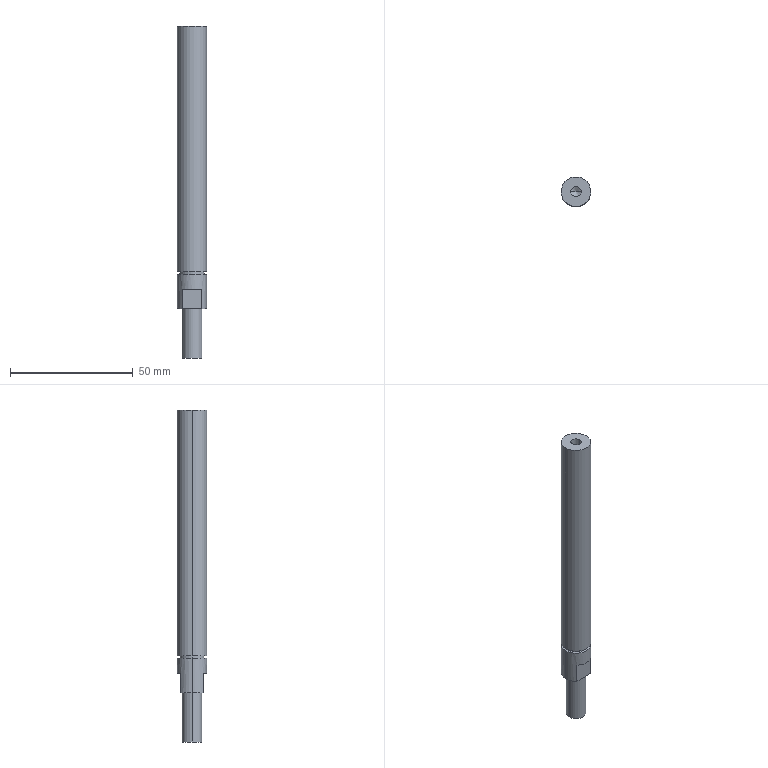Component | SolidWorks | GuideWheelAssembly2-1_RollerAxis1-1 | 1 solid | 21 faces | box 12 x 12 x 135 mm | volume 13669 mm3 | cylinder 10 | plane 9 | cone 2 | commonest cylinder face diameters 12 x4 8 x2 10 x2 4.2 x2
build123d program:
from build123d import *

# Parameters (mm, degrees)
SKETCH1_R             = 6
BOSS_EXTRUDE1_DEPTH   = 115
SKETCH3_R             = 4
BOSS_EXTRUDE2_DEPTH   = 20
CUT_EXTRUDE7_START    = -8
CUT_EXTRUDE7_DEPTH    = 8
M5_TAPPED_HOLE1_D     = 4.2
M5_TAPPED_HOLE1_DEPTH = 12.4
M5_TAPPED_HOLE1_TIP   = 1.262
SKETCH20_W            = 1
SKETCH20_H            = 1


with BuildPart() as part:
    # Sketch1 → Boss-Extrude1 (new body)
    with BuildSketch(Plane(origin=(0, 0, 0), x_dir=(1, 0, 0), z_dir=(0, 1, 0))):
        with Locations(Location((0, 0, 0), (0, 0, 270))):
            Circle(SKETCH1_R)
    extrude(amount=BOSS_EXTRUDE1_DEPTH)

    # Sketch3 → Boss-Extrude2 (add)
    with BuildSketch(Plane(origin=(0, 115, 0), x_dir=(1, 0, 0), z_dir=(0, 1, 0))):
        with Locations(Location((0, 0, 0), (0, 0, 270))):
            Circle(SKETCH3_R)
    extrude(amount=BOSS_EXTRUDE2_DEPTH)

    # Sketch17 → Cut-Extrude7 (cut)
    with BuildSketch(Plane(origin=(0, 115, 0), x_dir=(1, 0, 0), z_dir=(0, 1, 0)).offset(CUT_EXTRUDE7_START)):
        with BuildLine():
            Line((-4.5, 3.969), (-4.5, -3.969))
            ThreePointArc((-4.5, -3.969), (-6, 0), (-4.5, 3.969))
        make_face()
        with BuildLine():
            Line((4.5, 3.969), (4.5, -3.969))
            ThreePointArc((4.5, -3.969), (6, 0), (4.5, 3.969))
        make_face()
    extrude(amount=CUT_EXTRUDE7_DEPTH, mode=Mode.SUBTRACT)

    # M5 Tapped Hole1
    with Locations(Plane(origin=(0, 0, 0), x_dir=(-1, 0, 0), z_dir=(0, -1, 0))):
        with Locations((0, 0)):
            Hole(M5_TAPPED_HOLE1_D / 2, depth=M5_TAPPED_HOLE1_DEPTH)
            with Locations((0, 0, -(M5_TAPPED_HOLE1_DEPTH + M5_TAPPED_HOLE1_TIP / 2))):  # 118° drill point
                Cone(0, M5_TAPPED_HOLE1_D / 2, M5_TAPPED_HOLE1_TIP, mode=Mode.SUBTRACT)

    # Sketch20 → Cut-Revolve1 (revolve, cut)
    with BuildSketch(Plane(origin=(0, 0, 0), x_dir=(0, 0, -1), z_dir=(1, 0, 0)), mode=Mode.PRIVATE) as cut_revolve1_sk:
        with Locations((5.5, 100.5)):
            Rectangle(SKETCH20_W, SKETCH20_H)
    revolve(cut_revolve1_sk.sketch.rotate(Axis((0, 135, 0), (0, -1, 0)), 311.41), axis=Axis((0, 135, 0), (0, -1, 0)), mode=Mode.SUBTRACT)


solid = part.part

# Placed as in the assembly
solid = solid.moved(Location((-479.97, -65, 117), (-90, 90, 0)))
STEP:
#1=CARTESIAN_POINT('',(-18.66,-2.559,0.07874));
#2=VERTEX_POINT('',#1);
#3=CARTESIAN_POINT('',(-18.74,-2.736,0.07874));
#4=VERTEX_POINT('',#3);
#5=CARTESIAN_POINT('',(-18.896,-2.559,0.07874));
#6=DIRECTION('',(0.,0.,-1.));
#7=DIRECTION('',(1.,0.,-0.));
#8=AXIS2_PLACEMENT_3D('',#5,#6,#7);
#9=CIRCLE('',#8,0.2362);
#10=EDGE_CURVE('',#2,#4,#9,.T.);
#11=ORIENTED_EDGE('',*,*,#10,.F.);
#12=CARTESIAN_POINT('',(-18.66,-2.559,0.6299));
#13=VERTEX_POINT('',#12);
#14=CARTESIAN_POINT('',(-18.66,-2.559,0.07874));
#15=DIRECTION('',(-0.,-0.,1.));
#16=VECTOR('',#15,39.37);
#17=LINE('',#14,#16);
#18=EDGE_CURVE('',#2,#13,#17,.T.);
#19=ORIENTED_EDGE('',*,*,#18,.T.);
#20=CARTESIAN_POINT('',(-19.133,-2.559,0.6299));
#21=VERTEX_POINT('',#20);
#22=CARTESIAN_POINT('',(-18.896,-2.559,0.6299));
#23=DIRECTION('',(0.,0.,-1.));
#24=DIRECTION('',(1.,0.,0.));
#25=AXIS2_PLACEMENT_3D('',#22,#23,#24);
#26=CIRCLE('',#25,0.2362);
#27=EDGE_CURVE('',#13,#21,#26,.T.);
#28=ORIENTED_EDGE('',*,*,#27,.T.);
#29=CARTESIAN_POINT('',(-19.133,-2.559,0.07874));
#30=VERTEX_POINT('',#29);
#31=CARTESIAN_POINT('',(-19.133,-2.559,0.07874));
#32=DIRECTION('',(-0.,-0.,1.));
#33=VECTOR('',#32,39.37);
#34=LINE('',#31,#33);
#35=EDGE_CURVE('',#30,#21,#34,.T.);
#36=ORIENTED_EDGE('',*,*,#35,.F.);
#37=CARTESIAN_POINT('',(-19.053,-2.736,0.07874));
#38=VERTEX_POINT('',#37);
#39=CARTESIAN_POINT('',(-18.896,-2.559,0.07874));
#40=DIRECTION('',(0.,0.,-1.));
#41=DIRECTION('',(1.,0.,-0.));
#42=AXIS2_PLACEMENT_3D('',#39,#40,#41);
#43=CIRCLE('',#42,0.2362);
#44=EDGE_CURVE('',#38,#30,#43,.T.);
#45=ORIENTED_EDGE('',*,*,#44,.F.);
#46=CARTESIAN_POINT('',(-19.053,-2.736,0.3937));
#47=VERTEX_POINT('',#46);
#48=CARTESIAN_POINT('',(-19.053,-2.736,0.3937));
#49=DIRECTION('',(0.,0.,-1.));
#50=VECTOR('',#49,39.37);
#51=LINE('',#48,#50);
#52=EDGE_CURVE('',#47,#38,#51,.T.);
#53=ORIENTED_EDGE('',*,*,#52,.F.);
#54=CARTESIAN_POINT('',(-18.74,-2.736,0.3937));
#55=VERTEX_POINT('',#54);
#56=CARTESIAN_POINT('',(-18.896,-2.559,0.3937));
#57=DIRECTION('',(0.,0.,-1.));
#58=DIRECTION('',(1.,0.,0.));
#59=AXIS2_PLACEMENT_3D('',#56,#57,#58);
#60=CIRCLE('',#59,0.2362);
#61=EDGE_CURVE('',#55,#47,#60,.T.);
#62=ORIENTED_EDGE('',*,*,#61,.F.);
#63=CARTESIAN_POINT('',(-18.74,-2.736,0.3937));
#64=DIRECTION('',(0.,0.,-1.));
#65=VECTOR('',#64,39.37);
#66=LINE('',#63,#65);
#67=EDGE_CURVE('',#55,#4,#66,.T.);
#68=ORIENTED_EDGE('',*,*,#67,.T.);
#69=EDGE_LOOP('',(#11,#19,#28,#36,#45,#53,#62,#68));
#70=FACE_OUTER_BOUND('',#69,.T.);
#71=CARTESIAN_POINT('',(-18.896,-2.559,0.07874));
#72=DIRECTION('',(-0.,-0.,1.));
#73=DIRECTION('',(-1.,0.,0.));
#74=AXIS2_PLACEMENT_3D('',#71,#72,#73);
#75=CYLINDRICAL_SURFACE('',#74,0.2362);
#76=ADVANCED_FACE('',(#70),#75,.T.);
#77=CARTESIAN_POINT('',(-18.739,-2.559,-0.7087));
#78=VERTEX_POINT('',#77);
#79=CARTESIAN_POINT('',(-19.054,-2.559,-0.7087));
#80=VERTEX_POINT('',#79);
#81=CARTESIAN_POINT('',(-18.896,-2.559,-0.7087));
#82=DIRECTION('',(0.,0.,-1.));
#83=DIRECTION('',(1.,0.,0.));
#84=AXIS2_PLACEMENT_3D('',#81,#82,#83);
#85=CIRCLE('',#84,0.1575);
#86=EDGE_CURVE('',#78,#80,#85,.T.);
#87=ORIENTED_EDGE('',*,*,#86,.F.);
#88=CARTESIAN_POINT('',(-18.739,-2.559,0.07874));
#89=VERTEX_POINT('',#88);
#90=CARTESIAN_POINT('',(-18.739,-2.559,-0.7087));
#91=DIRECTION('',(-0.,-0.,1.));
#92=VECTOR('',#91,39.37);
#93=LINE('',#90,#92);
#94=EDGE_CURVE('',#78,#89,#93,.T.);
#95=ORIENTED_EDGE('',*,*,#94,.T.);
#96=CARTESIAN_POINT('',(-19.054,-2.559,0.07874));
#97=VERTEX_POINT('',#96);
#98=CARTESIAN_POINT('',(-18.896,-2.559,0.07874));
#99=DIRECTION('',(0.,0.,-1.));
#100=DIRECTION('',(1.,0.,-0.));
#101=AXIS2_PLACEMENT_3D('',#98,#99,#100);
#102=CIRCLE('',#101,0.1575);
#103=EDGE_CURVE('',#89,#97,#102,.T.);
#104=ORIENTED_EDGE('',*,*,#103,.T.);
#105=CARTESIAN_POINT('',(-19.054,-2.559,-0.7087));
#106=DIRECTION('',(-0.,-0.,1.));
#107=VECTOR('',#106,39.37);
#108=LINE('',#105,#107);
#109=EDGE_CURVE('',#80,#97,#108,.T.);
#110=ORIENTED_EDGE('',*,*,#109,.F.);
#111=EDGE_LOOP('',(#87,#95,#104,#110));
#112=FACE_OUTER_BOUND('',#111,.T.);
#113=CARTESIAN_POINT('',(-18.896,-2.559,-0.7087));
#114=DIRECTION('',(-0.,-0.,1.));
#115=DIRECTION('',(-1.,0.,0.));
#116=AXIS2_PLACEMENT_3D('',#113,#114,#115);
#117=CYLINDRICAL_SURFACE('',#116,0.1575);
#118=ADVANCED_FACE('',(#112),#117,.T.);
#119=CARTESIAN_POINT('',(-18.7,-2.559,0.6693));
#120=VERTEX_POINT('',#119);
#121=CARTESIAN_POINT('',(-19.093,-2.559,0.6693));
#122=VERTEX_POINT('',#121);
#123=CARTESIAN_POINT('',(-18.896,-2.559,0.6693));
#124=DIRECTION('',(0.,0.,-1.));
#125=DIRECTION('',(1.,0.,0.));
#126=AXIS2_PLACEMENT_3D('',#123,#124,#125);
#127=CIRCLE('',#126,0.1969);
#128=EDGE_CURVE('',#120,#122,#127,.T.);
#129=ORIENTED_EDGE('',*,*,#128,.T.);
#130=CARTESIAN_POINT('',(-19.093,-2.559,0.6299));
#131=VERTEX_POINT('',#130);
#132=CARTESIAN_POINT('',(-19.093,-2.559,-0.7087));
#133=DIRECTION('',(0.,0.,-1.));
#134=VECTOR('',#133,39.37);
#135=LINE('',#132,#134);
#136=EDGE_CURVE('',#122,#131,#135,.T.);
#137=ORIENTED_EDGE('',*,*,#136,.T.);
#138=CARTESIAN_POINT('',(-18.7,-2.559,0.6299));
#139=VERTEX_POINT('',#138);
#140=CARTESIAN_POINT('',(-18.896,-2.559,0.6299));
#141=DIRECTION('',(0.,0.,-1.));
#142=DIRECTION('',(1.,0.,0.));
#143=AXIS2_PLACEMENT_3D('',#140,#141,#142);
#144=CIRCLE('',#143,0.1969);
#145=EDGE_CURVE('',#139,#131,#144,.T.);
#146=ORIENTED_EDGE('',*,*,#145,.F.);
#147=CARTESIAN_POINT('',(-18.7,-2.559,-0.7087));
#148=DIRECTION('',(0.,0.,-1.));
#149=VECTOR('',#148,39.37);
#150=LINE('',#147,#149);
#151=EDGE_CURVE('',#120,#139,#150,.T.);
#152=ORIENTED_EDGE('',*,*,#151,.F.);
#153=EDGE_LOOP('',(#129,#137,#146,#152));
#154=FACE_OUTER_BOUND('',#153,.T.);
#155=CARTESIAN_POINT('',(-18.896,-2.559,-0.7087));
#156=DIRECTION('',(0.,0.,-1.));
#157=DIRECTION('',(1.,0.,0.));
#158=AXIS2_PLACEMENT_3D('',#155,#156,#157);
#159=CYLINDRICAL_SURFACE('',#158,0.1969);
#160=ADVANCED_FACE('',(#154),#159,.T.);
#161=CARTESIAN_POINT('',(-18.814,-2.559,4.118));
#162=VERTEX_POINT('',#161);
#163=CARTESIAN_POINT('',(-18.979,-2.559,4.118));
#164=VERTEX_POINT('',#163);
#165=CARTESIAN_POINT('',(-18.896,-2.559,4.118));
#166=DIRECTION('',(-0.,-0.,1.));
#167=DIRECTION('',(-1.,0.,0.));
#168=AXIS2_PLACEMENT_3D('',#165,#166,#167);
#169=CIRCLE('',#168,0.08268);
#170=EDGE_CURVE('',#162,#164,#169,.T.);
#171=ORIENTED_EDGE('',*,*,#170,.F.);
#172=CARTESIAN_POINT('',(-18.814,-2.559,4.606));
#173=VERTEX_POINT('',#172);
#174=CARTESIAN_POINT('',(-18.814,-2.559,4.606));
#175=DIRECTION('',(-0.,-0.,1.));
#176=VECTOR('',#175,39.37);
#177=LINE('',#174,#176);
#178=EDGE_CURVE('',#162,#173,#177,.T.);
#179=ORIENTED_EDGE('',*,*,#178,.T.);
#180=CARTESIAN_POINT('',(-18.979,-2.559,4.606));
#181=VERTEX_POINT('',#180);
#182=CARTESIAN_POINT('',(-18.896,-2.559,4.606));
#183=DIRECTION('',(-0.,-0.,1.));
#184=DIRECTION('',(-1.,0.,0.));
#185=AXIS2_PLACEMENT_3D('',#182,#183,#184);
#186=CIRCLE('',#185,0.08268);
#187=EDGE_CURVE('',#173,#181,#186,.T.);
#188=ORIENTED_EDGE('',*,*,#187,.T.);
#189=CARTESIAN_POINT('',(-18.979,-2.559,4.606));
#190=DIRECTION('',(-0.,-0.,1.));
#191=VECTOR('',#190,39.37);
#192=LINE('',#189,#191);
#193=EDGE_CURVE('',#164,#181,#192,.T.);
#194=ORIENTED_EDGE('',*,*,#193,.F.);
#195=EDGE_LOOP('',(#171,#179,#188,#194));
#196=FACE_OUTER_BOUND('',#195,.T.);
#197=CARTESIAN_POINT('',(-18.896,-2.559,4.606));
#198=DIRECTION('',(-0.,-0.,1.));
#199=DIRECTION('',(-1.,0.,0.));
#200=AXIS2_PLACEMENT_3D('',#197,#198,#199);
#201=CYLINDRICAL_SURFACE('',#200,0.08268);
#202=ADVANCED_FACE('',(#196),#201,.F.);
#203=CARTESIAN_POINT('',(-18.896,-2.559,4.068));
#204=VERTEX_POINT('',#203);
#205=CARTESIAN_POINT('',(-18.979,-2.559,4.118));
#206=DIRECTION('',(-0.8572,-0.,0.515));
#207=VECTOR('',#206,39.37);
#208=LINE('',#205,#207);
#209=EDGE_CURVE('',#204,#164,#208,.T.);
#210=ORIENTED_EDGE('',*,*,#209,.F.);
#211=CARTESIAN_POINT('',(-18.814,-2.559,4.118));
#212=DIRECTION('',(0.8572,0.,0.515));
#213=VECTOR('',#212,39.37);
#214=LINE('',#211,#213);
#215=EDGE_CURVE('',#204,#162,#214,.T.);
#216=ORIENTED_EDGE('',*,*,#215,.T.);
#217=ORIENTED_EDGE('',*,*,#170,.T.);
#218=EDGE_LOOP('',(#210,#216,#217));
#219=FACE_OUTER_BOUND('',#218,.T.);
#220=CARTESIAN_POINT('',(-18.896,-2.559,4.118));
#221=DIRECTION('',(-0.,-0.,1.));
#222=DIRECTION('',(-1.,0.,0.));
#223=AXIS2_PLACEMENT_3D('',#220,#221,#222);
#224=CONICAL_SURFACE('',#223,0.08268,1.03);
#225=ADVANCED_FACE('',(#219),#224,.F.);
#226=CARTESIAN_POINT('',(-18.66,-2.559,0.6693));
#227=VERTEX_POINT('',#226);
#228=CARTESIAN_POINT('',(-19.133,-2.559,0.6693));
#229=VERTEX_POINT('',#228);
#230=CARTESIAN_POINT('',(-18.896,-2.559,0.6693));
#231=DIRECTION('',(0.,0.,-1.));
#232=DIRECTION('',(1.,0.,0.));
#233=AXIS2_PLACEMENT_3D('',#230,#231,#232);
#234=CIRCLE('',#233,0.2362);
#235=EDGE_CURVE('',#227,#229,#234,.T.);
#236=ORIENTED_EDGE('',*,*,#235,.F.);
#237=CARTESIAN_POINT('',(-18.66,-2.559,4.606));
#238=VERTEX_POINT('',#237);
#239=CARTESIAN_POINT('',(-18.66,-2.559,0.07874));
#240=DIRECTION('',(-0.,-0.,1.));
#241=VECTOR('',#240,39.37);
#242=LINE('',#239,#241);
#243=EDGE_CURVE('',#227,#238,#242,.T.);
#244=ORIENTED_EDGE('',*,*,#243,.T.);
#245=CARTESIAN_POINT('',(-19.133,-2.559,4.606));
#246=VERTEX_POINT('',#245);
#247=CARTESIAN_POINT('',(-18.896,-2.559,4.606));
#248=DIRECTION('',(0.,0.,-1.));
#249=DIRECTION('',(1.,0.,0.));
#250=AXIS2_PLACEMENT_3D('',#247,#248,#249);
#251=CIRCLE('',#250,0.2362);
#252=EDGE_CURVE('',#238,#246,#251,.T.);
#253=ORIENTED_EDGE('',*,*,#252,.T.);
#254=CARTESIAN_POINT('',(-19.133,-2.559,0.07874));
#255=DIRECTION('',(-0.,-0.,1.));
#256=VECTOR('',#255,39.37);
#257=LINE('',#254,#256);
#258=EDGE_CURVE('',#229,#246,#257,.T.);
#259=ORIENTED_EDGE('',*,*,#258,.F.);
#260=EDGE_LOOP('',(#236,#244,#253,#259));
#261=FACE_OUTER_BOUND('',#260,.T.);
#262=CARTESIAN_POINT('',(-18.896,-2.559,0.07874));
#263=DIRECTION('',(-0.,-0.,1.));
#264=DIRECTION('',(-1.,0.,0.));
#265=AXIS2_PLACEMENT_3D('',#262,#263,#264);
#266=CYLINDRICAL_SURFACE('',#265,0.2362);
#267=ADVANCED_FACE('',(#261),#266,.T.);
#268=ORIENTED_EDGE('',*,*,#243,.F.);
#269=CARTESIAN_POINT('',(-18.896,-2.559,0.6693));
#270=DIRECTION('',(0.,0.,-1.));
#271=DIRECTION('',(1.,0.,0.));
#272=AXIS2_PLACEMENT_3D('',#269,#270,#271);
#273=CIRCLE('',#272,0.2362);
#274=EDGE_CURVE('',#229,#227,#273,.T.);
#275=ORIENTED_EDGE('',*,*,#274,.F.);
#276=ORIENTED_EDGE('',*,*,#258,.T.);
#277=CARTESIAN_POINT('',(-18.896,-2.559,4.606));
#278=DIRECTION('',(0.,0.,-1.));
#279=DIRECTION('',(1.,0.,0.));
#280=AXIS2_PLACEMENT_3D('',#277,#278,#279);
#281=CIRCLE('',#280,0.2362);
#282=EDGE_CURVE('',#246,#238,#281,.T.);
#283=ORIENTED_EDGE('',*,*,#282,.T.);
#284=EDGE_LOOP('',(#268,#275,#276,#283));
#285=FACE_OUTER_BOUND('',#284,.T.);
#286=CARTESIAN_POINT('',(-18.896,-2.559,0.07874));
#287=DIRECTION('',(-0.,-0.,1.));
#288=DIRECTION('',(-1.,0.,0.));
#289=AXIS2_PLACEMENT_3D('',#286,#287,#288);
#290=CYLINDRICAL_SURFACE('',#289,0.2362);
#291=ADVANCED_FACE('',(#285),#290,.T.);
#292=CARTESIAN_POINT('',(-18.896,-2.559,4.606));
#293=DIRECTION('',(-0.,-0.,1.));
#294=DIRECTION('',(-1.,0.,0.));
#295=AXIS2_PLACEMENT_3D('',#292,#293,#294);
#296=CIRCLE('',#295,0.08268);
#297=EDGE_CURVE('',#181,#173,#296,.T.);
#298=ORIENTED_EDGE('',*,*,#297,.F.);
#299=ORIENTED_EDGE('',*,*,#187,.F.);
#300=EDGE_LOOP('',(#298,#299));
#301=FACE_BOUND('',#300,.T.);
#302=ORIENTED_EDGE('',*,*,#282,.F.);
#303=ORIENTED_EDGE('',*,*,#252,.F.);
#304=EDGE_LOOP('',(#302,#303));
#305=FACE_OUTER_BOUND('',#304,.T.);
#306=CARTESIAN_POINT('',(-18.896,-2.559,4.606));
#307=DIRECTION('',(-0.,0.,-1.));
#308=DIRECTION('',(1.,0.,-0.));
#309=AXIS2_PLACEMENT_3D('',#306,#307,#308);
#310=PLANE('',#309);
#311=ADVANCED_FACE('',(#301,#305),#310,.F.);
#312=ORIENTED_EDGE('',*,*,#215,.F.);
#313=ORIENTED_EDGE('',*,*,#209,.T.);
#314=CARTESIAN_POINT('',(-18.896,-2.559,4.118));
#315=DIRECTION('',(-0.,-0.,1.));
#316=DIRECTION('',(-1.,0.,0.));
#317=AXIS2_PLACEMENT_3D('',#314,#315,#316);
#318=CIRCLE('',#317,0.08268);
#319=EDGE_CURVE('',#164,#162,#318,.T.);
#320=ORIENTED_EDGE('',*,*,#319,.T.);
#321=EDGE_LOOP('',(#312,#313,#320));
#322=FACE_OUTER_BOUND('',#321,.T.);
#323=CARTESIAN_POINT('',(-18.896,-2.559,4.118));
#324=DIRECTION('',(-0.,-0.,1.));
#325=DIRECTION('',(-1.,0.,0.));
#326=AXIS2_PLACEMENT_3D('',#323,#324,#325);
#327=CONICAL_SURFACE('',#326,0.08268,1.03);
#328=ADVANCED_FACE('',(#322),#327,.F.);
#329=ORIENTED_EDGE('',*,*,#178,.F.);
#330=ORIENTED_EDGE('',*,*,#319,.F.);
#331=ORIENTED_EDGE('',*,*,#193,.T.);
#332=ORIENTED_EDGE('',*,*,#297,.T.);
#333=EDGE_LOOP('',(#329,#330,#331,#332));
#334=FACE_OUTER_BOUND('',#333,.T.);
#335=CARTESIAN_POINT('',(-18.896,-2.559,4.606));
#336=DIRECTION('',(-0.,-0.,1.));
#337=DIRECTION('',(-1.,0.,0.));
#338=AXIS2_PLACEMENT_3D('',#335,#336,#337);
#339=CYLINDRICAL_SURFACE('',#338,0.08268);
#340=ADVANCED_FACE('',(#334),#339,.F.);
#341=ORIENTED_EDGE('',*,*,#274,.T.);
#342=ORIENTED_EDGE('',*,*,#235,.T.);
#343=EDGE_LOOP('',(#341,#342));
#344=FACE_OUTER_BOUND('',#343,.T.);
#345=ORIENTED_EDGE('',*,*,#128,.F.);
#346=CARTESIAN_POINT('',(-18.896,-2.559,0.6693));
#347=DIRECTION('',(0.,0.,-1.));
#348=DIRECTION('',(1.,0.,0.));
#349=AXIS2_PLACEMENT_3D('',#346,#347,#348);
#350=CIRCLE('',#349,0.1969);
#351=EDGE_CURVE('',#122,#120,#350,.T.);
#352=ORIENTED_EDGE('',*,*,#351,.F.);
#353=EDGE_LOOP('',(#345,#352));
#354=FACE_BOUND('',#353,.T.);
#355=CARTESIAN_POINT('',(-19.133,-2.559,0.6693));
#356=DIRECTION('',(-0.,0.,-1.));
#357=DIRECTION('',(1.,0.,-0.));
#358=AXIS2_PLACEMENT_3D('',#355,#356,#357);
#359=PLANE('',#358);
#360=ADVANCED_FACE('',(#344,#354),#359,.T.);
#361=ORIENTED_EDGE('',*,*,#136,.F.);
#362=ORIENTED_EDGE('',*,*,#351,.T.);
#363=ORIENTED_EDGE('',*,*,#151,.T.);
#364=CARTESIAN_POINT('',(-18.896,-2.559,0.6299));
#365=DIRECTION('',(0.,0.,-1.));
#366=DIRECTION('',(1.,0.,0.));
#367=AXIS2_PLACEMENT_3D('',#364,#365,#366);
#368=CIRCLE('',#367,0.1969);
#369=EDGE_CURVE('',#131,#139,#368,.T.);
#370=ORIENTED_EDGE('',*,*,#369,.F.);
#371=EDGE_LOOP('',(#361,#362,#363,#370));
#372=FACE_OUTER_BOUND('',#371,.T.);
#373=CARTESIAN_POINT('',(-18.896,-2.559,-0.7087));
#374=DIRECTION('',(0.,0.,-1.));
#375=DIRECTION('',(1.,0.,0.));
#376=AXIS2_PLACEMENT_3D('',#373,#374,#375);
#377=CYLINDRICAL_SURFACE('',#376,0.1969);
#378=ADVANCED_FACE('',(#372),#377,.T.);
#379=ORIENTED_EDGE('',*,*,#145,.T.);
#380=ORIENTED_EDGE('',*,*,#369,.T.);
#381=EDGE_LOOP('',(#379,#380));
#382=FACE_BOUND('',#381,.T.);
#383=CARTESIAN_POINT('',(-18.896,-2.559,0.6299));
#384=DIRECTION('',(0.,0.,-1.));
#385=DIRECTION('',(1.,0.,0.));
#386=AXIS2_PLACEMENT_3D('',#383,#384,#385);
#387=CIRCLE('',#386,0.2362);
#388=EDGE_CURVE('',#21,#13,#387,.T.);
#389=ORIENTED_EDGE('',*,*,#388,.F.);
#390=ORIENTED_EDGE('',*,*,#27,.F.);
#391=EDGE_LOOP('',(#389,#390));
#392=FACE_OUTER_BOUND('',#391,.T.);
#393=CARTESIAN_POINT('',(-19.133,-2.559,0.6299));
#394=DIRECTION('',(0.,-0.,1.));
#395=DIRECTION('',(-1.,-0.,0.));
#396=AXIS2_PLACEMENT_3D('',#393,#394,#395);
#397=PLANE('',#396);
#398=ADVANCED_FACE('',(#382,#392),#397,.T.);
#399=CARTESIAN_POINT('',(-18.896,-2.559,-0.7087));
#400=DIRECTION('',(0.,0.,-1.));
#401=DIRECTION('',(1.,0.,0.));
#402=AXIS2_PLACEMENT_3D('',#399,#400,#401);
#403=CIRCLE('',#402,0.1575);
#404=EDGE_CURVE('',#80,#78,#403,.T.);
#405=ORIENTED_EDGE('',*,*,#404,.T.);
#406=ORIENTED_EDGE('',*,*,#86,.T.);
#407=EDGE_LOOP('',(#405,#406));
#408=FACE_OUTER_BOUND('',#407,.T.);
#409=CARTESIAN_POINT('',(-18.896,-2.559,-0.7087));
#410=DIRECTION('',(-0.,0.,-1.));
#411=DIRECTION('',(1.,0.,-0.));
#412=AXIS2_PLACEMENT_3D('',#409,#410,#411);
#413=PLANE('',#412);
#414=ADVANCED_FACE('',(#408),#413,.T.);
#415=ORIENTED_EDGE('',*,*,#94,.F.);
#416=ORIENTED_EDGE('',*,*,#404,.F.);
#417=ORIENTED_EDGE('',*,*,#109,.T.);
#418=CARTESIAN_POINT('',(-18.896,-2.559,0.07874));
#419=DIRECTION('',(0.,0.,-1.));
#420=DIRECTION('',(1.,0.,-0.));
#421=AXIS2_PLACEMENT_3D('',#418,#419,#420);
#422=CIRCLE('',#421,0.1575);
#423=EDGE_CURVE('',#97,#89,#422,.T.);
#424=ORIENTED_EDGE('',*,*,#423,.T.);
#425=EDGE_LOOP('',(#415,#416,#417,#424));
#426=FACE_OUTER_BOUND('',#425,.T.);
#427=CARTESIAN_POINT('',(-18.896,-2.559,-0.7087));
#428=DIRECTION('',(-0.,-0.,1.));
#429=DIRECTION('',(-1.,0.,0.));
#430=AXIS2_PLACEMENT_3D('',#427,#428,#429);
#431=CYLINDRICAL_SURFACE('',#430,0.1575);
#432=ADVANCED_FACE('',(#426),#431,.T.);
#433=ORIENTED_EDGE('',*,*,#61,.T.);
#434=CARTESIAN_POINT('',(-19.053,-2.736,0.3937));
#435=DIRECTION('',(1.,0.,-0.));
#436=VECTOR('',#435,39.37);
#437=LINE('',#434,#436);
#438=EDGE_CURVE('',#47,#55,#437,.T.);
#439=ORIENTED_EDGE('',*,*,#438,.T.);
#440=EDGE_LOOP('',(#433,#439));
#441=FACE_OUTER_BOUND('',#440,.T.);
#442=CARTESIAN_POINT('',(-18.896,-2.559,0.3937));
#443=DIRECTION('',(-0.,0.,-1.));
#444=DIRECTION('',(1.,0.,-0.));
#445=AXIS2_PLACEMENT_3D('',#442,#443,#444);
#446=PLANE('',#445);
#447=ADVANCED_FACE('',(#441),#446,.T.);
#448=CARTESIAN_POINT('',(-19.053,-2.736,0.07874));
#449=DIRECTION('',(1.,0.,-0.));
#450=VECTOR('',#449,39.37);
#451=LINE('',#448,#450);
#452=EDGE_CURVE('',#38,#4,#451,.T.);
#453=ORIENTED_EDGE('',*,*,#452,.T.);
#454=ORIENTED_EDGE('',*,*,#67,.F.);
#455=ORIENTED_EDGE('',*,*,#438,.F.);
#456=ORIENTED_EDGE('',*,*,#52,.T.);
#457=EDGE_LOOP('',(#453,#454,#455,#456));
#458=FACE_OUTER_BOUND('',#457,.T.);
#459=CARTESIAN_POINT('',(-19.053,-2.736,0.3937));
#460=DIRECTION('',(-0.,1.,0.));
#461=DIRECTION('',(1.,0.,-0.));
#462=AXIS2_PLACEMENT_3D('',#459,#460,#461);
#463=PLANE('',#462);
#464=ADVANCED_FACE('',(#458),#463,.F.);
#465=CARTESIAN_POINT('',(-19.053,-2.382,0.3937));
#466=VERTEX_POINT('',#465);
#467=CARTESIAN_POINT('',(-18.74,-2.382,0.3937));
#468=VERTEX_POINT('',#467);
#469=CARTESIAN_POINT('',(-18.896,-2.559,0.3937));
#470=DIRECTION('',(0.,0.,-1.));
#471=DIRECTION('',(1.,0.,0.));
#472=AXIS2_PLACEMENT_3D('',#469,#470,#471);
#473=CIRCLE('',#472,0.2362);
#474=EDGE_CURVE('',#466,#468,#473,.T.);
#475=ORIENTED_EDGE('',*,*,#474,.T.);
#476=CARTESIAN_POINT('',(-19.053,-2.382,0.3937));
#477=DIRECTION('',(-1.,-0.,0.));
#478=VECTOR('',#477,39.37);
#479=LINE('',#476,#478);
#480=EDGE_CURVE('',#468,#466,#479,.T.);
#481=ORIENTED_EDGE('',*,*,#480,.T.);
#482=EDGE_LOOP('',(#475,#481));
#483=FACE_OUTER_BOUND('',#482,.T.);
#484=CARTESIAN_POINT('',(-18.896,-2.559,0.3937));
#485=DIRECTION('',(-0.,0.,-1.));
#486=DIRECTION('',(1.,0.,-0.));
#487=AXIS2_PLACEMENT_3D('',#484,#485,#486);
#488=PLANE('',#487);
#489=ADVANCED_FACE('',(#483),#488,.T.);
#490=CARTESIAN_POINT('',(-18.74,-2.382,0.07874));
#491=VERTEX_POINT('',#490);
#492=CARTESIAN_POINT('',(-19.053,-2.382,0.07874));
#493=VERTEX_POINT('',#492);
#494=CARTESIAN_POINT('',(-19.053,-2.382,0.07874));
#495=DIRECTION('',(-1.,-0.,0.));
#496=VECTOR('',#495,39.37);
#497=LINE('',#494,#496);
#498=EDGE_CURVE('',#491,#493,#497,.T.);
#499=ORIENTED_EDGE('',*,*,#498,.T.);
#500=CARTESIAN_POINT('',(-19.053,-2.382,0.3937));
#501=DIRECTION('',(0.,0.,-1.));
#502=VECTOR('',#501,39.37);
#503=LINE('',#500,#502);
#504=EDGE_CURVE('',#466,#493,#503,.T.);
#505=ORIENTED_EDGE('',*,*,#504,.F.);
#506=ORIENTED_EDGE('',*,*,#480,.F.);
#507=CARTESIAN_POINT('',(-18.74,-2.382,0.3937));
#508=DIRECTION('',(0.,0.,-1.));
#509=VECTOR('',#508,39.37);
#510=LINE('',#507,#509);
#511=EDGE_CURVE('',#468,#491,#510,.T.);
#512=ORIENTED_EDGE('',*,*,#511,.T.);
#513=EDGE_LOOP('',(#499,#505,#506,#512));
#514=FACE_OUTER_BOUND('',#513,.T.);
#515=CARTESIAN_POINT('',(-19.053,-2.382,0.3937));
#516=DIRECTION('',(0.,-1.,-0.));
#517=DIRECTION('',(-1.,-0.,0.));
#518=AXIS2_PLACEMENT_3D('',#515,#516,#517);
#519=PLANE('',#518);
#520=ADVANCED_FACE('',(#514),#519,.F.);
#521=ORIENTED_EDGE('',*,*,#498,.F.);
#522=CARTESIAN_POINT('',(-18.896,-2.559,0.07874));
#523=DIRECTION('',(0.,0.,-1.));
#524=DIRECTION('',(1.,0.,-0.));
#525=AXIS2_PLACEMENT_3D('',#522,#523,#524);
#526=CIRCLE('',#525,0.2362);
#527=EDGE_CURVE('',#491,#2,#526,.T.);
#528=ORIENTED_EDGE('',*,*,#527,.T.);
#529=ORIENTED_EDGE('',*,*,#10,.T.);
#530=ORIENTED_EDGE('',*,*,#452,.F.);
#531=ORIENTED_EDGE('',*,*,#44,.T.);
#532=CARTESIAN_POINT('',(-18.896,-2.559,0.07874));
#533=DIRECTION('',(0.,0.,-1.));
#534=DIRECTION('',(1.,0.,-0.));
#535=AXIS2_PLACEMENT_3D('',#532,#533,#534);
#536=CIRCLE('',#535,0.2362);
#537=EDGE_CURVE('',#30,#493,#536,.T.);
#538=ORIENTED_EDGE('',*,*,#537,.T.);
#539=EDGE_LOOP('',(#521,#528,#529,#530,#531,#538));
#540=FACE_OUTER_BOUND('',#539,.T.);
#541=ORIENTED_EDGE('',*,*,#423,.F.);
#542=ORIENTED_EDGE('',*,*,#103,.F.);
#543=EDGE_LOOP('',(#541,#542));
#544=FACE_BOUND('',#543,.T.);
#545=CARTESIAN_POINT('',(-18.896,-2.559,0.07874));
#546=DIRECTION('',(-0.,0.,-1.));
#547=DIRECTION('',(1.,0.,-0.));
#548=AXIS2_PLACEMENT_3D('',#545,#546,#547);
#549=PLANE('',#548);
#550=ADVANCED_FACE('',(#540,#544),#549,.T.);
#551=ORIENTED_EDGE('',*,*,#18,.F.);
#552=ORIENTED_EDGE('',*,*,#527,.F.);
#553=ORIENTED_EDGE('',*,*,#511,.F.);
#554=ORIENTED_EDGE('',*,*,#474,.F.);
#555=ORIENTED_EDGE('',*,*,#504,.T.);
#556=ORIENTED_EDGE('',*,*,#537,.F.);
#557=ORIENTED_EDGE('',*,*,#35,.T.);
#558=ORIENTED_EDGE('',*,*,#388,.T.);
#559=EDGE_LOOP('',(#551,#552,#553,#554,#555,#556,#557,#558));
#560=FACE_OUTER_BOUND('',#559,.T.);
#561=CARTESIAN_POINT('',(-18.896,-2.559,0.07874));
#562=DIRECTION('',(-0.,-0.,1.));
#563=DIRECTION('',(-1.,0.,0.));
#564=AXIS2_PLACEMENT_3D('',#561,#562,#563);
#565=CYLINDRICAL_SURFACE('',#564,0.2362);
#566=ADVANCED_FACE('',(#560),#565,.T.);
#567=CLOSED_SHELL('',(#76,#118,#160,#202,#225,#267,#291,#311,#328,#340,#360,#378,#398,#414,#432,#447,#464,#489,#520,#550,#566));
#568=MANIFOLD_SOLID_BREP('',#567);
#569=CARTESIAN_POINT('',(0.,0.,0.));
#570=DIRECTION('',(0.,0.,1.));
#571=DIRECTION('',(1.,0.,0.));
#572=AXIS2_PLACEMENT_3D('',#569,#570,#571);
#573=(LENGTH_UNIT()NAMED_UNIT(*)SI_UNIT($,.METRE.));
#574=LENGTH_MEASURE_WITH_UNIT(LENGTH_MEASURE(0.0254),#573);
#575=DIMENSIONAL_EXPONENTS(1.,0.,0.,0.,0.,0.,0.);
#576=(CONVERSION_BASED_UNIT('',#574)LENGTH_UNIT()NAMED_UNIT(#575));
#577=UNCERTAINTY_MEASURE_WITH_UNIT(LENGTH_MEASURE(0.00001),#576,'','');
#578=(NAMED_UNIT(*)PLANE_ANGLE_UNIT()SI_UNIT($,.RADIAN.));
#579=(NAMED_UNIT(*)SI_UNIT($,.STERADIAN.)SOLID_ANGLE_UNIT());
#580=(GEOMETRIC_REPRESENTATION_CONTEXT(3)GLOBAL_UNCERTAINTY_ASSIGNED_CONTEXT((#577))GLOBAL_UNIT_ASSIGNED_CONTEXT((#576,#578,#579))REPRESENTATION_CONTEXT('',''));
#581=ADVANCED_BREP_SHAPE_REPRESENTATION('',(#568,#572),#580);
#582=COLOUR_RGB('',0.7922,0.8196,0.9333);
#583=FILL_AREA_STYLE_COLOUR('',#582);
#584=FILL_AREA_STYLE('',(#583));
#585=SURFACE_STYLE_FILL_AREA(#584);
#586=SURFACE_SIDE_STYLE('',(#585));
#587=SURFACE_STYLE_USAGE(.BOTH.,#586);
#588=PRESENTATION_STYLE_ASSIGNMENT((#587));
#589=STYLED_ITEM('',(#588),#568);
#590=(LENGTH_UNIT()NAMED_UNIT(*)SI_UNIT($,.METRE.));
#591=LENGTH_MEASURE_WITH_UNIT(LENGTH_MEASURE(0.0254),#590);
#592=DIMENSIONAL_EXPONENTS(1.,0.,0.,0.,0.,0.,0.);
#593=(CONVERSION_BASED_UNIT('',#591)LENGTH_UNIT()NAMED_UNIT(#592));
#594=UNCERTAINTY_MEASURE_WITH_UNIT(LENGTH_MEASURE(0.00001),#593,'','');
#595=(NAMED_UNIT(*)PLANE_ANGLE_UNIT()SI_UNIT($,.RADIAN.));
#596=(NAMED_UNIT(*)SI_UNIT($,.STERADIAN.)SOLID_ANGLE_UNIT());
#597=(GEOMETRIC_REPRESENTATION_CONTEXT(3)GLOBAL_UNCERTAINTY_ASSIGNED_CONTEXT((#594))GLOBAL_UNIT_ASSIGNED_CONTEXT((#593,#595,#596))REPRESENTATION_CONTEXT('',''));
#598=MECHANICAL_DESIGN_GEOMETRIC_PRESENTATION_REPRESENTATION('',(#589),#597);
#599=PRESENTATION_LAYER_ASSIGNMENT('','',(#589));